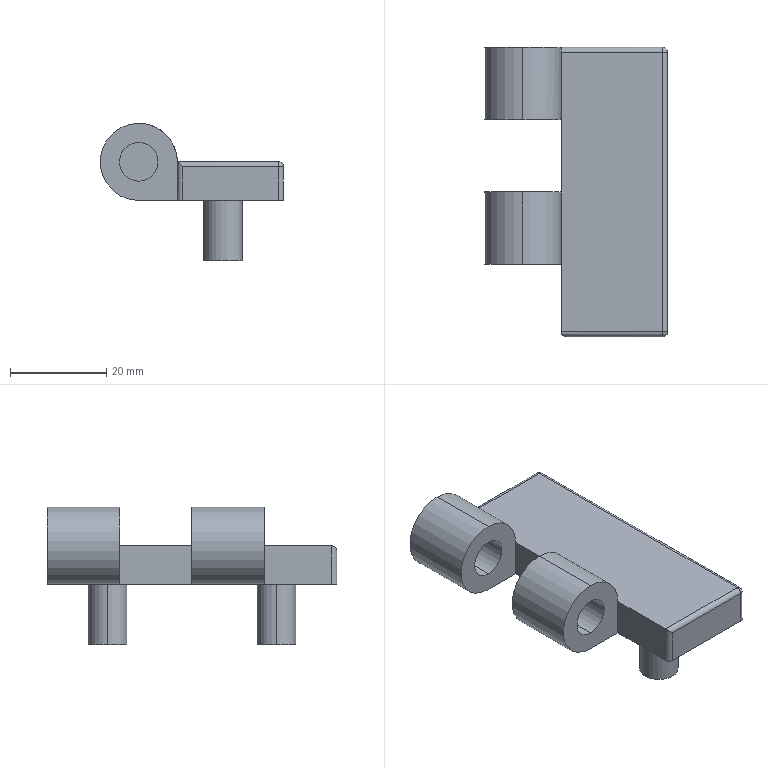Component | SolidWorks | DoorHinge1-1 | 1 solid | 33 faces | box 38 x 60 x 28.5 mm | volume 16826 mm3 | cylinder 18 | plane 13 | sphere 2 | commonest cylinder face diameters 8 x8 2 x6 16 x4
STEP:
#1=CARTESIAN_POINT('',(85.649,76.317,49.177));
#2=VERTEX_POINT('',#1);
#3=CARTESIAN_POINT('',(85.649,76.317,48.862));
#4=VERTEX_POINT('',#3);
#5=CARTESIAN_POINT('',(85.649,76.317,49.02));
#6=DIRECTION('',(-0.,-1.,0.));
#7=DIRECTION('',(0.,0.,-1.));
#8=AXIS2_PLACEMENT_3D('',#5,#6,#7);
#9=CIRCLE('',#8,0.1575);
#10=EDGE_CURVE('',#2,#4,#9,.T.);
#11=ORIENTED_EDGE('',*,*,#10,.F.);
#12=CARTESIAN_POINT('',(85.649,75.806,49.177));
#13=VERTEX_POINT('',#12);
#14=CARTESIAN_POINT('',(85.649,76.317,49.177));
#15=DIRECTION('',(-0.,-1.,0.));
#16=VECTOR('',#15,39.37);
#17=LINE('',#14,#16);
#18=EDGE_CURVE('',#2,#13,#17,.T.);
#19=ORIENTED_EDGE('',*,*,#18,.T.);
#20=CARTESIAN_POINT('',(85.649,75.806,48.862));
#21=VERTEX_POINT('',#20);
#22=CARTESIAN_POINT('',(85.649,75.806,49.02));
#23=DIRECTION('',(0.,1.,-0.));
#24=DIRECTION('',(-1.,0.,0.));
#25=AXIS2_PLACEMENT_3D('',#22,#23,#24);
#26=CIRCLE('',#25,0.1575);
#27=EDGE_CURVE('',#21,#13,#26,.T.);
#28=ORIENTED_EDGE('',*,*,#27,.F.);
#29=CARTESIAN_POINT('',(85.649,76.317,48.862));
#30=DIRECTION('',(-0.,-1.,0.));
#31=VECTOR('',#30,39.37);
#32=LINE('',#29,#31);
#33=EDGE_CURVE('',#4,#21,#32,.T.);
#34=ORIENTED_EDGE('',*,*,#33,.F.);
#35=EDGE_LOOP('',(#11,#19,#28,#34));
#36=FACE_OUTER_BOUND('',#35,.T.);
#37=CARTESIAN_POINT('',(85.649,76.317,49.02));
#38=DIRECTION('',(-0.,-1.,0.));
#39=DIRECTION('',(0.,0.,-1.));
#40=AXIS2_PLACEMENT_3D('',#37,#38,#39);
#41=CYLINDRICAL_SURFACE('',#40,0.1575);
#42=ADVANCED_FACE('',(#36),#41,.F.);
#43=CARTESIAN_POINT('',(86.495,75.904,48.213));
#44=VERTEX_POINT('',#43);
#45=CARTESIAN_POINT('',(86.18,75.904,48.213));
#46=VERTEX_POINT('',#45);
#47=CARTESIAN_POINT('',(86.338,75.904,48.213));
#48=DIRECTION('',(-0.,-0.,-1.));
#49=DIRECTION('',(1.,0.,0.));
#50=AXIS2_PLACEMENT_3D('',#47,#48,#49);
#51=CIRCLE('',#50,0.1575);
#52=EDGE_CURVE('',#44,#46,#51,.T.);
#53=ORIENTED_EDGE('',*,*,#52,.F.);
#54=CARTESIAN_POINT('',(86.495,75.904,48.705));
#55=VERTEX_POINT('',#54);
#56=CARTESIAN_POINT('',(86.495,75.904,48.213));
#57=DIRECTION('',(0.,0.,1.));
#58=VECTOR('',#57,39.37);
#59=LINE('',#56,#58);
#60=EDGE_CURVE('',#44,#55,#59,.T.);
#61=ORIENTED_EDGE('',*,*,#60,.T.);
#62=CARTESIAN_POINT('',(86.18,75.904,48.705));
#63=VERTEX_POINT('',#62);
#64=CARTESIAN_POINT('',(86.338,75.904,48.705));
#65=DIRECTION('',(-0.,-0.,-1.));
#66=DIRECTION('',(-1.,0.,0.));
#67=AXIS2_PLACEMENT_3D('',#64,#65,#66);
#68=CIRCLE('',#67,0.1575);
#69=EDGE_CURVE('',#55,#63,#68,.T.);
#70=ORIENTED_EDGE('',*,*,#69,.T.);
#71=CARTESIAN_POINT('',(86.18,75.904,48.213));
#72=DIRECTION('',(0.,0.,1.));
#73=VECTOR('',#72,39.37);
#74=LINE('',#71,#73);
#75=EDGE_CURVE('',#46,#63,#74,.T.);
#76=ORIENTED_EDGE('',*,*,#75,.F.);
#77=EDGE_LOOP('',(#53,#61,#70,#76));
#78=FACE_OUTER_BOUND('',#77,.T.);
#79=CARTESIAN_POINT('',(86.338,75.904,48.213));
#80=DIRECTION('',(0.,0.,1.));
#81=DIRECTION('',(-1.,0.,0.));
#82=AXIS2_PLACEMENT_3D('',#79,#80,#81);
#83=CYLINDRICAL_SURFACE('',#82,0.1575);
#84=ADVANCED_FACE('',(#78),#83,.T.);
#85=CARTESIAN_POINT('',(86.495,74.526,48.213));
#86=VERTEX_POINT('',#85);
#87=CARTESIAN_POINT('',(86.18,74.526,48.213));
#88=VERTEX_POINT('',#87);
#89=CARTESIAN_POINT('',(86.338,74.526,48.213));
#90=DIRECTION('',(-0.,-0.,-1.));
#91=DIRECTION('',(1.,0.,0.));
#92=AXIS2_PLACEMENT_3D('',#89,#90,#91);
#93=CIRCLE('',#92,0.1575);
#94=EDGE_CURVE('',#86,#88,#93,.T.);
#95=ORIENTED_EDGE('',*,*,#94,.F.);
#96=CARTESIAN_POINT('',(86.495,74.526,48.705));
#97=VERTEX_POINT('',#96);
#98=CARTESIAN_POINT('',(86.495,74.526,48.213));
#99=DIRECTION('',(0.,0.,1.));
#100=VECTOR('',#99,39.37);
#101=LINE('',#98,#100);
#102=EDGE_CURVE('',#86,#97,#101,.T.);
#103=ORIENTED_EDGE('',*,*,#102,.T.);
#104=CARTESIAN_POINT('',(86.18,74.526,48.705));
#105=VERTEX_POINT('',#104);
#106=CARTESIAN_POINT('',(86.338,74.526,48.705));
#107=DIRECTION('',(-0.,-0.,-1.));
#108=DIRECTION('',(-1.,0.,0.));
#109=AXIS2_PLACEMENT_3D('',#106,#107,#108);
#110=CIRCLE('',#109,0.1575);
#111=EDGE_CURVE('',#97,#105,#110,.T.);
#112=ORIENTED_EDGE('',*,*,#111,.T.);
#113=CARTESIAN_POINT('',(86.18,74.526,48.213));
#114=DIRECTION('',(0.,0.,1.));
#115=VECTOR('',#114,39.37);
#116=LINE('',#113,#115);
#117=EDGE_CURVE('',#88,#105,#116,.T.);
#118=ORIENTED_EDGE('',*,*,#117,.F.);
#119=EDGE_LOOP('',(#95,#103,#112,#118));
#120=FACE_OUTER_BOUND('',#119,.T.);
#121=CARTESIAN_POINT('',(86.338,74.526,48.213));
#122=DIRECTION('',(0.,0.,1.));
#123=DIRECTION('',(-1.,0.,0.));
#124=AXIS2_PLACEMENT_3D('',#121,#122,#123);
#125=CYLINDRICAL_SURFACE('',#124,0.1575);
#126=ADVANCED_FACE('',(#120),#125,.T.);
#127=CARTESIAN_POINT('',(85.649,75.215,49.177));
#128=VERTEX_POINT('',#127);
#129=CARTESIAN_POINT('',(85.649,75.215,48.862));
#130=VERTEX_POINT('',#129);
#131=CARTESIAN_POINT('',(85.649,75.215,49.02));
#132=DIRECTION('',(-0.,-1.,0.));
#133=DIRECTION('',(1.,0.,0.));
#134=AXIS2_PLACEMENT_3D('',#131,#132,#133);
#135=CIRCLE('',#134,0.1575);
#136=EDGE_CURVE('',#128,#130,#135,.T.);
#137=ORIENTED_EDGE('',*,*,#136,.F.);
#138=CARTESIAN_POINT('',(85.649,74.624,49.177));
#139=VERTEX_POINT('',#138);
#140=CARTESIAN_POINT('',(85.649,76.317,49.177));
#141=DIRECTION('',(-0.,-1.,0.));
#142=VECTOR('',#141,39.37);
#143=LINE('',#140,#142);
#144=EDGE_CURVE('',#128,#139,#143,.T.);
#145=ORIENTED_EDGE('',*,*,#144,.T.);
#146=CARTESIAN_POINT('',(85.649,74.624,48.862));
#147=VERTEX_POINT('',#146);
#148=CARTESIAN_POINT('',(85.649,74.624,49.02));
#149=DIRECTION('',(0.,1.,-0.));
#150=DIRECTION('',(0.,0.,-1.));
#151=AXIS2_PLACEMENT_3D('',#148,#149,#150);
#152=CIRCLE('',#151,0.1575);
#153=EDGE_CURVE('',#147,#139,#152,.T.);
#154=ORIENTED_EDGE('',*,*,#153,.F.);
#155=CARTESIAN_POINT('',(85.649,76.317,48.862));
#156=DIRECTION('',(-0.,-1.,0.));
#157=VECTOR('',#156,39.37);
#158=LINE('',#155,#157);
#159=EDGE_CURVE('',#130,#147,#158,.T.);
#160=ORIENTED_EDGE('',*,*,#159,.F.);
#161=EDGE_LOOP('',(#137,#145,#154,#160));
#162=FACE_OUTER_BOUND('',#161,.T.);
#163=CARTESIAN_POINT('',(85.649,76.317,49.02));
#164=DIRECTION('',(-0.,-1.,0.));
#165=DIRECTION('',(0.,0.,-1.));
#166=AXIS2_PLACEMENT_3D('',#163,#164,#165);
#167=CYLINDRICAL_SURFACE('',#166,0.1575);
#168=ADVANCED_FACE('',(#162),#167,.F.);
#169=CARTESIAN_POINT('',(85.649,75.806,49.335));
#170=VERTEX_POINT('',#169);
#171=CARTESIAN_POINT('',(85.649,75.806,48.705));
#172=VERTEX_POINT('',#171);
#173=CARTESIAN_POINT('',(85.649,75.806,49.02));
#174=DIRECTION('',(-0.,-1.,0.));
#175=DIRECTION('',(-1.,0.,0.));
#176=AXIS2_PLACEMENT_3D('',#173,#174,#175);
#177=CIRCLE('',#176,0.315);
#178=EDGE_CURVE('',#170,#172,#177,.T.);
#179=ORIENTED_EDGE('',*,*,#178,.F.);
#180=CARTESIAN_POINT('',(85.649,76.396,49.335));
#181=VERTEX_POINT('',#180);
#182=CARTESIAN_POINT('',(85.649,74.034,49.335));
#183=DIRECTION('',(0.,1.,-0.));
#184=VECTOR('',#183,39.37);
#185=LINE('',#182,#184);
#186=EDGE_CURVE('',#170,#181,#185,.T.);
#187=ORIENTED_EDGE('',*,*,#186,.T.);
#188=CARTESIAN_POINT('',(85.649,76.396,48.705));
#189=VERTEX_POINT('',#188);
#190=CARTESIAN_POINT('',(85.649,76.396,49.02));
#191=DIRECTION('',(-0.,-1.,0.));
#192=DIRECTION('',(0.,0.,-1.));
#193=AXIS2_PLACEMENT_3D('',#190,#191,#192);
#194=CIRCLE('',#193,0.315);
#195=EDGE_CURVE('',#181,#189,#194,.T.);
#196=ORIENTED_EDGE('',*,*,#195,.T.);
#197=CARTESIAN_POINT('',(85.649,74.034,48.705));
#198=DIRECTION('',(0.,1.,-0.));
#199=VECTOR('',#198,39.37);
#200=LINE('',#197,#199);
#201=EDGE_CURVE('',#172,#189,#200,.T.);
#202=ORIENTED_EDGE('',*,*,#201,.F.);
#203=EDGE_LOOP('',(#179,#187,#196,#202));
#204=FACE_OUTER_BOUND('',#203,.T.);
#205=CARTESIAN_POINT('',(85.649,74.034,49.02));
#206=DIRECTION('',(0.,1.,-0.));
#207=DIRECTION('',(0.,0.,1.));
#208=AXIS2_PLACEMENT_3D('',#205,#206,#207);
#209=CYLINDRICAL_SURFACE('',#208,0.315);
#210=ADVANCED_FACE('',(#204),#209,.T.);
#211=CARTESIAN_POINT('',(85.649,74.624,49.335));
#212=VERTEX_POINT('',#211);
#213=CARTESIAN_POINT('',(85.649,74.624,48.705));
#214=VERTEX_POINT('',#213);
#215=CARTESIAN_POINT('',(85.649,74.624,49.02));
#216=DIRECTION('',(-0.,-1.,0.));
#217=DIRECTION('',(0.,0.,-1.));
#218=AXIS2_PLACEMENT_3D('',#215,#216,#217);
#219=CIRCLE('',#218,0.315);
#220=EDGE_CURVE('',#212,#214,#219,.T.);
#221=ORIENTED_EDGE('',*,*,#220,.F.);
#222=CARTESIAN_POINT('',(85.649,75.215,49.335));
#223=VERTEX_POINT('',#222);
#224=CARTESIAN_POINT('',(85.649,74.034,49.335));
#225=DIRECTION('',(0.,1.,-0.));
#226=VECTOR('',#225,39.37);
#227=LINE('',#224,#226);
#228=EDGE_CURVE('',#212,#223,#227,.T.);
#229=ORIENTED_EDGE('',*,*,#228,.T.);
#230=CARTESIAN_POINT('',(85.649,75.215,48.705));
#231=VERTEX_POINT('',#230);
#232=CARTESIAN_POINT('',(85.649,75.215,49.02));
#233=DIRECTION('',(0.,1.,-0.));
#234=DIRECTION('',(1.,0.,0.));
#235=AXIS2_PLACEMENT_3D('',#232,#233,#234);
#236=CIRCLE('',#235,0.315);
#237=EDGE_CURVE('',#231,#223,#236,.T.);
#238=ORIENTED_EDGE('',*,*,#237,.F.);
#239=CARTESIAN_POINT('',(85.649,74.034,48.705));
#240=DIRECTION('',(0.,1.,-0.));
#241=VECTOR('',#240,39.37);
#242=LINE('',#239,#241);
#243=EDGE_CURVE('',#214,#231,#242,.T.);
#244=ORIENTED_EDGE('',*,*,#243,.F.);
#245=EDGE_LOOP('',(#221,#229,#238,#244));
#246=FACE_OUTER_BOUND('',#245,.T.);
#247=CARTESIAN_POINT('',(85.649,74.034,49.02));
#248=DIRECTION('',(0.,1.,-0.));
#249=DIRECTION('',(0.,0.,1.));
#250=AXIS2_PLACEMENT_3D('',#247,#248,#249);
#251=CYLINDRICAL_SURFACE('',#250,0.315);
#252=ADVANCED_FACE('',(#246),#251,.T.);
#253=CARTESIAN_POINT('',(86.338,74.526,48.705));
#254=DIRECTION('',(-0.,-0.,-1.));
#255=DIRECTION('',(-1.,0.,0.));
#256=AXIS2_PLACEMENT_3D('',#253,#254,#255);
#257=CIRCLE('',#256,0.1575);
#258=EDGE_CURVE('',#105,#97,#257,.T.);
#259=ORIENTED_EDGE('',*,*,#258,.F.);
#260=ORIENTED_EDGE('',*,*,#111,.F.);
#261=EDGE_LOOP('',(#259,#260));
#262=FACE_BOUND('',#261,.T.);
#263=CARTESIAN_POINT('',(86.338,75.904,48.705));
#264=DIRECTION('',(-0.,-0.,-1.));
#265=DIRECTION('',(-1.,0.,0.));
#266=AXIS2_PLACEMENT_3D('',#263,#264,#265);
#267=CIRCLE('',#266,0.1575);
#268=EDGE_CURVE('',#63,#55,#267,.T.);
#269=ORIENTED_EDGE('',*,*,#268,.F.);
#270=ORIENTED_EDGE('',*,*,#69,.F.);
#271=EDGE_LOOP('',(#269,#270));
#272=FACE_BOUND('',#271,.T.);
#273=CARTESIAN_POINT('',(86.79,76.396,48.705));
#274=VERTEX_POINT('',#273);
#275=CARTESIAN_POINT('',(84.813,76.396,48.705));
#276=DIRECTION('',(1.,-0.,-0.));
#277=VECTOR('',#276,39.37);
#278=LINE('',#275,#277);
#279=EDGE_CURVE('',#189,#274,#278,.T.);
#280=ORIENTED_EDGE('',*,*,#279,.T.);
#281=CARTESIAN_POINT('',(86.83,76.357,48.705));
#282=VERTEX_POINT('',#281);
#283=CARTESIAN_POINT('',(86.79,76.357,48.705));
#284=DIRECTION('',(-0.,-0.,-1.));
#285=DIRECTION('',(-1.,0.,0.));
#286=AXIS2_PLACEMENT_3D('',#283,#284,#285);
#287=CIRCLE('',#286,0.03937);
#288=EDGE_CURVE('',#274,#282,#287,.T.);
#289=ORIENTED_EDGE('',*,*,#288,.T.);
#290=CARTESIAN_POINT('',(86.83,74.073,48.705));
#291=VERTEX_POINT('',#290);
#292=CARTESIAN_POINT('',(86.83,74.034,48.705));
#293=DIRECTION('',(0.,1.,-0.));
#294=VECTOR('',#293,39.37);
#295=LINE('',#292,#294);
#296=EDGE_CURVE('',#291,#282,#295,.T.);
#297=ORIENTED_EDGE('',*,*,#296,.F.);
#298=CARTESIAN_POINT('',(86.79,74.034,48.705));
#299=VERTEX_POINT('',#298);
#300=CARTESIAN_POINT('',(86.79,74.073,48.705));
#301=DIRECTION('',(-0.,-0.,-1.));
#302=DIRECTION('',(-1.,0.,0.));
#303=AXIS2_PLACEMENT_3D('',#300,#301,#302);
#304=CIRCLE('',#303,0.03937);
#305=EDGE_CURVE('',#291,#299,#304,.T.);
#306=ORIENTED_EDGE('',*,*,#305,.T.);
#307=CARTESIAN_POINT('',(86.003,74.034,48.705));
#308=VERTEX_POINT('',#307);
#309=CARTESIAN_POINT('',(84.813,74.034,48.705));
#310=DIRECTION('',(1.,-0.,-0.));
#311=VECTOR('',#310,39.37);
#312=LINE('',#309,#311);
#313=EDGE_CURVE('',#308,#299,#312,.T.);
#314=ORIENTED_EDGE('',*,*,#313,.F.);
#315=CARTESIAN_POINT('',(85.963,74.073,48.705));
#316=VERTEX_POINT('',#315);
#317=CARTESIAN_POINT('',(86.003,74.073,48.705));
#318=DIRECTION('',(-0.,-0.,-1.));
#319=DIRECTION('',(-1.,0.,0.));
#320=AXIS2_PLACEMENT_3D('',#317,#318,#319);
#321=CIRCLE('',#320,0.03937);
#322=EDGE_CURVE('',#308,#316,#321,.T.);
#323=ORIENTED_EDGE('',*,*,#322,.T.);
#324=CARTESIAN_POINT('',(85.963,74.624,48.705));
#325=VERTEX_POINT('',#324);
#326=CARTESIAN_POINT('',(85.963,77.404,48.705));
#327=DIRECTION('',(0.,1.,-0.));
#328=VECTOR('',#327,39.37);
#329=LINE('',#326,#328);
#330=EDGE_CURVE('',#316,#325,#329,.T.);
#331=ORIENTED_EDGE('',*,*,#330,.T.);
#332=CARTESIAN_POINT('',(86.136,74.624,48.705));
#333=DIRECTION('',(-1.,0.,0.));
#334=VECTOR('',#333,39.37);
#335=LINE('',#332,#334);
#336=EDGE_CURVE('',#325,#214,#335,.T.);
#337=ORIENTED_EDGE('',*,*,#336,.T.);
#338=ORIENTED_EDGE('',*,*,#243,.T.);
#339=CARTESIAN_POINT('',(85.963,75.215,48.705));
#340=VERTEX_POINT('',#339);
#341=CARTESIAN_POINT('',(85.334,75.215,48.705));
#342=DIRECTION('',(1.,-0.,-0.));
#343=VECTOR('',#342,39.37);
#344=LINE('',#341,#343);
#345=EDGE_CURVE('',#231,#340,#344,.T.);
#346=ORIENTED_EDGE('',*,*,#345,.T.);
#347=CARTESIAN_POINT('',(85.963,75.806,48.705));
#348=VERTEX_POINT('',#347);
#349=CARTESIAN_POINT('',(85.963,75.215,48.705));
#350=DIRECTION('',(0.,1.,-0.));
#351=VECTOR('',#350,39.37);
#352=LINE('',#349,#351);
#353=EDGE_CURVE('',#340,#348,#352,.T.);
#354=ORIENTED_EDGE('',*,*,#353,.T.);
#355=CARTESIAN_POINT('',(85.963,75.806,48.705));
#356=DIRECTION('',(-1.,0.,0.));
#357=VECTOR('',#356,39.37);
#358=LINE('',#355,#357);
#359=EDGE_CURVE('',#348,#172,#358,.T.);
#360=ORIENTED_EDGE('',*,*,#359,.T.);
#361=ORIENTED_EDGE('',*,*,#201,.T.);
#362=EDGE_LOOP('',(#280,#289,#297,#306,#314,#323,#331,#337,#338,#346,#354,#360,#361));
#363=FACE_OUTER_BOUND('',#362,.T.);
#364=CARTESIAN_POINT('',(84.813,74.034,48.705));
#365=DIRECTION('',(0.,0.,1.));
#366=DIRECTION('',(-1.,0.,0.));
#367=AXIS2_PLACEMENT_3D('',#364,#365,#366);
#368=PLANE('',#367);
#369=ADVANCED_FACE('',(#262,#272,#363),#368,.F.);
#370=ORIENTED_EDGE('',*,*,#228,.F.);
#371=CARTESIAN_POINT('',(85.963,74.624,49.02));
#372=VERTEX_POINT('',#371);
#373=CARTESIAN_POINT('',(85.649,74.624,49.02));
#374=DIRECTION('',(-0.,-1.,0.));
#375=DIRECTION('',(0.,0.,-1.));
#376=AXIS2_PLACEMENT_3D('',#373,#374,#375);
#377=CIRCLE('',#376,0.315);
#378=EDGE_CURVE('',#372,#212,#377,.T.);
#379=ORIENTED_EDGE('',*,*,#378,.F.);
#380=CARTESIAN_POINT('',(85.963,75.215,49.02));
#381=VERTEX_POINT('',#380);
#382=CARTESIAN_POINT('',(85.963,74.034,49.02));
#383=DIRECTION('',(0.,1.,-0.));
#384=VECTOR('',#383,39.37);
#385=LINE('',#382,#384);
#386=EDGE_CURVE('',#372,#381,#385,.T.);
#387=ORIENTED_EDGE('',*,*,#386,.T.);
#388=CARTESIAN_POINT('',(85.649,75.215,49.02));
#389=DIRECTION('',(0.,1.,-0.));
#390=DIRECTION('',(1.,0.,0.));
#391=AXIS2_PLACEMENT_3D('',#388,#389,#390);
#392=CIRCLE('',#391,0.315);
#393=EDGE_CURVE('',#223,#381,#392,.T.);
#394=ORIENTED_EDGE('',*,*,#393,.F.);
#395=EDGE_LOOP('',(#370,#379,#387,#394));
#396=FACE_OUTER_BOUND('',#395,.T.);
#397=CARTESIAN_POINT('',(85.649,74.034,49.02));
#398=DIRECTION('',(0.,1.,-0.));
#399=DIRECTION('',(0.,0.,1.));
#400=AXIS2_PLACEMENT_3D('',#397,#398,#399);
#401=CYLINDRICAL_SURFACE('',#400,0.315);
#402=ADVANCED_FACE('',(#396),#401,.T.);
#403=ORIENTED_EDGE('',*,*,#186,.F.);
#404=CARTESIAN_POINT('',(85.963,75.806,49.02));
#405=VERTEX_POINT('',#404);
#406=CARTESIAN_POINT('',(85.649,75.806,49.02));
#407=DIRECTION('',(-0.,-1.,0.));
#408=DIRECTION('',(-1.,0.,0.));
#409=AXIS2_PLACEMENT_3D('',#406,#407,#408);
#410=CIRCLE('',#409,0.315);
#411=EDGE_CURVE('',#405,#170,#410,.T.);
#412=ORIENTED_EDGE('',*,*,#411,.F.);
#413=CARTESIAN_POINT('',(85.963,76.357,49.02));
#414=VERTEX_POINT('',#413);
#415=CARTESIAN_POINT('',(85.963,74.034,49.02));
#416=DIRECTION('',(0.,1.,-0.));
#417=VECTOR('',#416,39.37);
#418=LINE('',#415,#417);
#419=EDGE_CURVE('',#405,#414,#418,.T.);
#420=ORIENTED_EDGE('',*,*,#419,.T.);
#421=CARTESIAN_POINT('',(85.961,76.396,48.981));
#422=VERTEX_POINT('',#421);
#423=CARTESIAN_POINT('',(85.963,76.357,49.02));
#424=CARTESIAN_POINT('',(85.963,76.362,49.02));
#425=CARTESIAN_POINT('',(85.963,76.367,49.019));
#426=CARTESIAN_POINT('',(85.963,76.377,49.015));
#427=CARTESIAN_POINT('',(85.963,76.381,49.012));
#428=CARTESIAN_POINT('',(85.963,76.388,49.005));
#429=CARTESIAN_POINT('',(85.963,76.391,49.));
#430=CARTESIAN_POINT('',(85.962,76.395,48.991));
#431=CARTESIAN_POINT('',(85.962,76.396,48.986));
#432=CARTESIAN_POINT('',(85.961,76.396,48.981));
#433=B_SPLINE_CURVE_WITH_KNOTS('',3,(#423,#424,#425,#426,#427,#428,#429,#430,#431,#432),.UNSPECIFIED.,.F.,.F.,(4,2,2,2,4),(0.,0.0003912,0.0007823,0.001173,0.001565),.UNSPECIFIED.);
#434=EDGE_CURVE('',#414,#422,#433,.T.);
#435=ORIENTED_EDGE('',*,*,#434,.T.);
#436=CARTESIAN_POINT('',(85.649,76.396,49.02));
#437=DIRECTION('',(-0.,-1.,0.));
#438=DIRECTION('',(0.,0.,-1.));
#439=AXIS2_PLACEMENT_3D('',#436,#437,#438);
#440=CIRCLE('',#439,0.315);
#441=EDGE_CURVE('',#422,#181,#440,.T.);
#442=ORIENTED_EDGE('',*,*,#441,.T.);
#443=EDGE_LOOP('',(#403,#412,#420,#435,#442));
#444=FACE_OUTER_BOUND('',#443,.T.);
#445=CARTESIAN_POINT('',(85.649,74.034,49.02));
#446=DIRECTION('',(0.,1.,-0.));
#447=DIRECTION('',(0.,0.,1.));
#448=AXIS2_PLACEMENT_3D('',#445,#446,#447);
#449=CYLINDRICAL_SURFACE('',#448,0.315);
#450=ADVANCED_FACE('',(#444),#449,.T.);
#451=ORIENTED_EDGE('',*,*,#144,.F.);
#452=CARTESIAN_POINT('',(85.649,75.215,49.02));
#453=DIRECTION('',(-0.,-1.,0.));
#454=DIRECTION('',(1.,0.,0.));
#455=AXIS2_PLACEMENT_3D('',#452,#453,#454);
#456=CIRCLE('',#455,0.1575);
#457=EDGE_CURVE('',#130,#128,#456,.T.);
#458=ORIENTED_EDGE('',*,*,#457,.F.);
#459=ORIENTED_EDGE('',*,*,#159,.T.);
#460=CARTESIAN_POINT('',(85.649,74.624,49.02));
#461=DIRECTION('',(0.,1.,-0.));
#462=DIRECTION('',(0.,0.,-1.));
#463=AXIS2_PLACEMENT_3D('',#460,#461,#462);
#464=CIRCLE('',#463,0.1575);
#465=EDGE_CURVE('',#139,#147,#464,.T.);
#466=ORIENTED_EDGE('',*,*,#465,.F.);
#467=EDGE_LOOP('',(#451,#458,#459,#466));
#468=FACE_OUTER_BOUND('',#467,.T.);
#469=CARTESIAN_POINT('',(85.649,76.317,49.02));
#470=DIRECTION('',(-0.,-1.,0.));
#471=DIRECTION('',(0.,0.,-1.));
#472=AXIS2_PLACEMENT_3D('',#469,#470,#471);
#473=CYLINDRICAL_SURFACE('',#472,0.1575);
#474=ADVANCED_FACE('',(#468),#473,.F.);
#475=CARTESIAN_POINT('',(86.79,74.034,48.981));
#476=VERTEX_POINT('',#475);
#477=CARTESIAN_POINT('',(86.003,74.034,48.981));
#478=VERTEX_POINT('',#477);
#479=CARTESIAN_POINT('',(85.963,74.034,48.981));
#480=DIRECTION('',(-1.,0.,0.));
#481=VECTOR('',#480,39.37);
#482=LINE('',#479,#481);
#483=EDGE_CURVE('',#476,#478,#482,.T.);
#484=ORIENTED_EDGE('',*,*,#483,.T.);
#485=CARTESIAN_POINT('',(86.003,74.034,49.02));
#486=DIRECTION('',(-0.,-0.,-1.));
#487=VECTOR('',#486,39.37);
#488=LINE('',#485,#487);
#489=EDGE_CURVE('',#478,#308,#488,.T.);
#490=ORIENTED_EDGE('',*,*,#489,.T.);
#491=ORIENTED_EDGE('',*,*,#313,.T.);
#492=CARTESIAN_POINT('',(86.79,74.034,49.02));
#493=DIRECTION('',(0.,0.,1.));
#494=VECTOR('',#493,39.37);
#495=LINE('',#492,#494);
#496=EDGE_CURVE('',#299,#476,#495,.T.);
#497=ORIENTED_EDGE('',*,*,#496,.T.);
#498=EDGE_LOOP('',(#484,#490,#491,#497));
#499=FACE_OUTER_BOUND('',#498,.T.);
#500=CARTESIAN_POINT('',(84.813,74.034,49.02));
#501=DIRECTION('',(-0.,-1.,0.));
#502=DIRECTION('',(-0.,-0.,-1.));
#503=AXIS2_PLACEMENT_3D('',#500,#501,#502);
#504=PLANE('',#503);
#505=ADVANCED_FACE('',(#499),#504,.T.);
#506=ORIENTED_EDGE('',*,*,#296,.T.);
#507=CARTESIAN_POINT('',(86.83,76.357,48.981));
#508=VERTEX_POINT('',#507);
#509=CARTESIAN_POINT('',(86.83,76.357,49.02));
#510=DIRECTION('',(0.,0.,1.));
#511=VECTOR('',#510,39.37);
#512=LINE('',#509,#511);
#513=EDGE_CURVE('',#282,#508,#512,.T.);
#514=ORIENTED_EDGE('',*,*,#513,.T.);
#515=CARTESIAN_POINT('',(86.83,74.073,48.981));
#516=VERTEX_POINT('',#515);
#517=CARTESIAN_POINT('',(86.83,74.034,48.981));
#518=DIRECTION('',(-0.,-1.,0.));
#519=VECTOR('',#518,39.37);
#520=LINE('',#517,#519);
#521=EDGE_CURVE('',#508,#516,#520,.T.);
#522=ORIENTED_EDGE('',*,*,#521,.T.);
#523=CARTESIAN_POINT('',(86.83,74.073,48.705));
#524=DIRECTION('',(-0.,-0.,-1.));
#525=VECTOR('',#524,39.37);
#526=LINE('',#523,#525);
#527=EDGE_CURVE('',#516,#291,#526,.T.);
#528=ORIENTED_EDGE('',*,*,#527,.T.);
#529=EDGE_LOOP('',(#506,#514,#522,#528));
#530=FACE_OUTER_BOUND('',#529,.T.);
#531=CARTESIAN_POINT('',(86.83,74.034,49.02));
#532=DIRECTION('',(-1.,0.,0.));
#533=DIRECTION('',(-0.,-0.,-1.));
#534=AXIS2_PLACEMENT_3D('',#531,#532,#533);
#535=PLANE('',#534);
#536=ADVANCED_FACE('',(#530),#535,.F.);
#537=CARTESIAN_POINT('',(85.963,74.073,49.02));
#538=VERTEX_POINT('',#537);
#539=CARTESIAN_POINT('',(85.963,74.034,49.02));
#540=DIRECTION('',(0.,1.,-0.));
#541=VECTOR('',#540,39.37);
#542=LINE('',#539,#541);
#543=EDGE_CURVE('',#538,#372,#542,.T.);
#544=ORIENTED_EDGE('',*,*,#543,.F.);
#545=CARTESIAN_POINT('',(86.79,74.073,49.02));
#546=VERTEX_POINT('',#545);
#547=CARTESIAN_POINT('',(86.83,74.073,49.02));
#548=DIRECTION('',(1.,-0.,-0.));
#549=VECTOR('',#548,39.37);
#550=LINE('',#547,#549);
#551=EDGE_CURVE('',#538,#546,#550,.T.);
#552=ORIENTED_EDGE('',*,*,#551,.T.);
#553=CARTESIAN_POINT('',(86.79,76.357,49.02));
#554=VERTEX_POINT('',#553);
#555=CARTESIAN_POINT('',(86.79,74.034,49.02));
#556=DIRECTION('',(0.,1.,-0.));
#557=VECTOR('',#556,39.37);
#558=LINE('',#555,#557);
#559=EDGE_CURVE('',#546,#554,#558,.T.);
#560=ORIENTED_EDGE('',*,*,#559,.T.);
#561=CARTESIAN_POINT('',(84.813,76.357,49.02));
#562=DIRECTION('',(-1.,0.,0.));
#563=VECTOR('',#562,39.37);
#564=LINE('',#561,#563);
#565=EDGE_CURVE('',#554,#414,#564,.T.);
#566=ORIENTED_EDGE('',*,*,#565,.T.);
#567=ORIENTED_EDGE('',*,*,#419,.F.);
#568=CARTESIAN_POINT('',(85.963,74.034,49.02));
#569=DIRECTION('',(0.,1.,-0.));
#570=VECTOR('',#569,39.37);
#571=LINE('',#568,#570);
#572=EDGE_CURVE('',#381,#405,#571,.T.);
#573=ORIENTED_EDGE('',*,*,#572,.F.);
#574=ORIENTED_EDGE('',*,*,#386,.F.);
#575=EDGE_LOOP('',(#544,#552,#560,#566,#567,#573,#574));
#576=FACE_OUTER_BOUND('',#575,.T.);
#577=CARTESIAN_POINT('',(84.813,74.034,49.02));
#578=DIRECTION('',(-0.,0.,-1.));
#579=DIRECTION('',(1.,-0.,-0.));
#580=AXIS2_PLACEMENT_3D('',#577,#578,#579);
#581=PLANE('',#580);
#582=ADVANCED_FACE('',(#576),#581,.F.);
#583=CARTESIAN_POINT('',(86.79,76.396,48.981));
#584=VERTEX_POINT('',#583);
#585=CARTESIAN_POINT('',(84.813,76.396,48.981));
#586=DIRECTION('',(1.,-0.,-0.));
#587=VECTOR('',#586,39.37);
#588=LINE('',#585,#587);
#589=EDGE_CURVE('',#422,#584,#588,.T.);
#590=ORIENTED_EDGE('',*,*,#589,.T.);
#591=CARTESIAN_POINT('',(86.79,76.396,49.02));
#592=DIRECTION('',(-0.,-0.,-1.));
#593=VECTOR('',#592,39.37);
#594=LINE('',#591,#593);
#595=EDGE_CURVE('',#584,#274,#594,.T.);
#596=ORIENTED_EDGE('',*,*,#595,.T.);
#597=ORIENTED_EDGE('',*,*,#279,.F.);
#598=ORIENTED_EDGE('',*,*,#195,.F.);
#599=ORIENTED_EDGE('',*,*,#441,.F.);
#600=EDGE_LOOP('',(#590,#596,#597,#598,#599));
#601=FACE_OUTER_BOUND('',#600,.T.);
#602=CARTESIAN_POINT('',(84.813,76.396,49.02));
#603=DIRECTION('',(-0.,-1.,0.));
#604=DIRECTION('',(-0.,-0.,-1.));
#605=AXIS2_PLACEMENT_3D('',#602,#603,#604);
#606=PLANE('',#605);
#607=ADVANCED_FACE('',(#601),#606,.F.);
#608=ORIENTED_EDGE('',*,*,#102,.F.);
#609=CARTESIAN_POINT('',(86.338,74.526,48.213));
#610=DIRECTION('',(-0.,-0.,-1.));
#611=DIRECTION('',(1.,0.,0.));
#612=AXIS2_PLACEMENT_3D('',#609,#610,#611);
#613=CIRCLE('',#612,0.1575);
#614=EDGE_CURVE('',#88,#86,#613,.T.);
#615=ORIENTED_EDGE('',*,*,#614,.F.);
#616=ORIENTED_EDGE('',*,*,#117,.T.);
#617=ORIENTED_EDGE('',*,*,#258,.T.);
#618=EDGE_LOOP('',(#608,#615,#616,#617));
#619=FACE_OUTER_BOUND('',#618,.T.);
#620=CARTESIAN_POINT('',(86.338,74.526,48.213));
#621=DIRECTION('',(0.,0.,1.));
#622=DIRECTION('',(-1.,0.,0.));
#623=AXIS2_PLACEMENT_3D('',#620,#621,#622);
#624=CYLINDRICAL_SURFACE('',#623,0.1575);
#625=ADVANCED_FACE('',(#619),#624,.T.);
#626=ORIENTED_EDGE('',*,*,#614,.T.);
#627=ORIENTED_EDGE('',*,*,#94,.T.);
#628=EDGE_LOOP('',(#626,#627));
#629=FACE_OUTER_BOUND('',#628,.T.);
#630=CARTESIAN_POINT('',(86.338,74.526,48.213));
#631=DIRECTION('',(-0.,-0.,-1.));
#632=DIRECTION('',(1.,-0.,-0.));
#633=AXIS2_PLACEMENT_3D('',#630,#631,#632);
#634=PLANE('',#633);
#635=ADVANCED_FACE('',(#629),#634,.T.);
#636=ORIENTED_EDGE('',*,*,#60,.F.);
#637=CARTESIAN_POINT('',(86.338,75.904,48.213));
#638=DIRECTION('',(-0.,-0.,-1.));
#639=DIRECTION('',(1.,0.,0.));
#640=AXIS2_PLACEMENT_3D('',#637,#638,#639);
#641=CIRCLE('',#640,0.1575);
#642=EDGE_CURVE('',#46,#44,#641,.T.);
#643=ORIENTED_EDGE('',*,*,#642,.F.);
#644=ORIENTED_EDGE('',*,*,#75,.T.);
#645=ORIENTED_EDGE('',*,*,#268,.T.);
#646=EDGE_LOOP('',(#636,#643,#644,#645));
#647=FACE_OUTER_BOUND('',#646,.T.);
#648=CARTESIAN_POINT('',(86.338,75.904,48.213));
#649=DIRECTION('',(0.,0.,1.));
#650=DIRECTION('',(-1.,0.,0.));
#651=AXIS2_PLACEMENT_3D('',#648,#649,#650);
#652=CYLINDRICAL_SURFACE('',#651,0.1575);
#653=ADVANCED_FACE('',(#647),#652,.T.);
#654=ORIENTED_EDGE('',*,*,#642,.T.);
#655=ORIENTED_EDGE('',*,*,#52,.T.);
#656=EDGE_LOOP('',(#654,#655));
#657=FACE_OUTER_BOUND('',#656,.T.);
#658=CARTESIAN_POINT('',(86.338,75.904,48.213));
#659=DIRECTION('',(-0.,-0.,-1.));
#660=DIRECTION('',(1.,-0.,-0.));
#661=AXIS2_PLACEMENT_3D('',#658,#659,#660);
#662=PLANE('',#661);
#663=ADVANCED_FACE('',(#657),#662,.T.);
#664=ORIENTED_EDGE('',*,*,#330,.F.);
#665=CARTESIAN_POINT('',(85.963,74.073,50.988));
#666=DIRECTION('',(0.,0.,1.));
#667=VECTOR('',#666,39.37);
#668=LINE('',#665,#667);
#669=EDGE_CURVE('',#316,#538,#668,.T.);
#670=ORIENTED_EDGE('',*,*,#669,.T.);
#671=ORIENTED_EDGE('',*,*,#543,.T.);
#672=CARTESIAN_POINT('',(85.963,74.624,50.988));
#673=DIRECTION('',(-0.,-0.,-1.));
#674=VECTOR('',#673,39.37);
#675=LINE('',#672,#674);
#676=EDGE_CURVE('',#372,#325,#675,.T.);
#677=ORIENTED_EDGE('',*,*,#676,.T.);
#678=EDGE_LOOP('',(#664,#670,#671,#677));
#679=FACE_OUTER_BOUND('',#678,.T.);
#680=CARTESIAN_POINT('',(85.963,77.404,50.988));
#681=DIRECTION('',(-1.,0.,0.));
#682=DIRECTION('',(-0.,-0.,-1.));
#683=AXIS2_PLACEMENT_3D('',#680,#681,#682);
#684=PLANE('',#683);
#685=ADVANCED_FACE('',(#679),#684,.T.);
#686=ORIENTED_EDGE('',*,*,#153,.T.);
#687=ORIENTED_EDGE('',*,*,#465,.T.);
#688=EDGE_LOOP('',(#686,#687));
#689=FACE_BOUND('',#688,.T.);
#690=ORIENTED_EDGE('',*,*,#378,.T.);
#691=ORIENTED_EDGE('',*,*,#220,.T.);
#692=ORIENTED_EDGE('',*,*,#336,.F.);
#693=ORIENTED_EDGE('',*,*,#676,.F.);
#694=EDGE_LOOP('',(#690,#691,#692,#693));
#695=FACE_OUTER_BOUND('',#694,.T.);
#696=CARTESIAN_POINT('',(86.136,74.624,50.988));
#697=DIRECTION('',(-0.,-1.,0.));
#698=DIRECTION('',(-0.,-0.,-1.));
#699=AXIS2_PLACEMENT_3D('',#696,#697,#698);
#700=PLANE('',#699);
#701=ADVANCED_FACE('',(#689,#695),#700,.T.);
#702=ORIENTED_EDGE('',*,*,#572,.T.);
#703=CARTESIAN_POINT('',(85.963,75.806,50.988));
#704=DIRECTION('',(-0.,-0.,-1.));
#705=VECTOR('',#704,39.37);
#706=LINE('',#703,#705);
#707=EDGE_CURVE('',#405,#348,#706,.T.);
#708=ORIENTED_EDGE('',*,*,#707,.T.);
#709=ORIENTED_EDGE('',*,*,#353,.F.);
#710=CARTESIAN_POINT('',(85.963,75.215,50.988));
#711=DIRECTION('',(-0.,-0.,-1.));
#712=VECTOR('',#711,39.37);
#713=LINE('',#710,#712);
#714=EDGE_CURVE('',#381,#340,#713,.T.);
#715=ORIENTED_EDGE('',*,*,#714,.F.);
#716=EDGE_LOOP('',(#702,#708,#709,#715));
#717=FACE_OUTER_BOUND('',#716,.T.);
#718=CARTESIAN_POINT('',(85.963,75.215,50.988));
#719=DIRECTION('',(-1.,0.,0.));
#720=DIRECTION('',(0.,1.,-0.));
#721=AXIS2_PLACEMENT_3D('',#718,#719,#720);
#722=PLANE('',#721);
#723=ADVANCED_FACE('',(#717),#722,.T.);
#724=ORIENTED_EDGE('',*,*,#457,.T.);
#725=ORIENTED_EDGE('',*,*,#136,.T.);
#726=EDGE_LOOP('',(#724,#725));
#727=FACE_BOUND('',#726,.T.);
#728=ORIENTED_EDGE('',*,*,#237,.T.);
#729=ORIENTED_EDGE('',*,*,#393,.T.);
#730=ORIENTED_EDGE('',*,*,#714,.T.);
#731=ORIENTED_EDGE('',*,*,#345,.F.);
#732=EDGE_LOOP('',(#728,#729,#730,#731));
#733=FACE_OUTER_BOUND('',#732,.T.);
#734=CARTESIAN_POINT('',(85.334,75.215,50.988));
#735=DIRECTION('',(0.,1.,-0.));
#736=DIRECTION('',(1.,-0.,-0.));
#737=AXIS2_PLACEMENT_3D('',#734,#735,#736);
#738=PLANE('',#737);
#739=ADVANCED_FACE('',(#727,#733),#738,.T.);
#740=ORIENTED_EDGE('',*,*,#27,.T.);
#741=CARTESIAN_POINT('',(85.649,75.806,49.02));
#742=DIRECTION('',(0.,1.,-0.));
#743=DIRECTION('',(-1.,0.,0.));
#744=AXIS2_PLACEMENT_3D('',#741,#742,#743);
#745=CIRCLE('',#744,0.1575);
#746=EDGE_CURVE('',#13,#21,#745,.T.);
#747=ORIENTED_EDGE('',*,*,#746,.T.);
#748=EDGE_LOOP('',(#740,#747));
#749=FACE_BOUND('',#748,.T.);
#750=ORIENTED_EDGE('',*,*,#411,.T.);
#751=ORIENTED_EDGE('',*,*,#178,.T.);
#752=ORIENTED_EDGE('',*,*,#359,.F.);
#753=ORIENTED_EDGE('',*,*,#707,.F.);
#754=EDGE_LOOP('',(#750,#751,#752,#753));
#755=FACE_OUTER_BOUND('',#754,.T.);
#756=CARTESIAN_POINT('',(85.963,75.806,50.988));
#757=DIRECTION('',(-0.,-1.,0.));
#758=DIRECTION('',(-1.,0.,0.));
#759=AXIS2_PLACEMENT_3D('',#756,#757,#758);
#760=PLANE('',#759);
#761=ADVANCED_FACE('',(#749,#755),#760,.T.);
#762=CARTESIAN_POINT('',(85.649,76.317,49.02));
#763=DIRECTION('',(-0.,-1.,0.));
#764=DIRECTION('',(0.,0.,-1.));
#765=AXIS2_PLACEMENT_3D('',#762,#763,#764);
#766=CIRCLE('',#765,0.1575);
#767=EDGE_CURVE('',#4,#2,#766,.T.);
#768=ORIENTED_EDGE('',*,*,#767,.T.);
#769=ORIENTED_EDGE('',*,*,#10,.T.);
#770=EDGE_LOOP('',(#768,#769));
#771=FACE_OUTER_BOUND('',#770,.T.);
#772=CARTESIAN_POINT('',(85.649,76.317,49.02));
#773=DIRECTION('',(-0.,-1.,0.));
#774=DIRECTION('',(-0.,-0.,-1.));
#775=AXIS2_PLACEMENT_3D('',#772,#773,#774);
#776=PLANE('',#775);
#777=ADVANCED_FACE('',(#771),#776,.T.);
#778=ORIENTED_EDGE('',*,*,#18,.F.);
#779=ORIENTED_EDGE('',*,*,#767,.F.);
#780=ORIENTED_EDGE('',*,*,#33,.T.);
#781=ORIENTED_EDGE('',*,*,#746,.F.);
#782=EDGE_LOOP('',(#778,#779,#780,#781));
#783=FACE_OUTER_BOUND('',#782,.T.);
#784=CARTESIAN_POINT('',(85.649,76.317,49.02));
#785=DIRECTION('',(-0.,-1.,0.));
#786=DIRECTION('',(0.,0.,-1.));
#787=AXIS2_PLACEMENT_3D('',#784,#785,#786);
#788=CYLINDRICAL_SURFACE('',#787,0.1575);
#789=ADVANCED_FACE('',(#783),#788,.F.);
#790=ORIENTED_EDGE('',*,*,#322,.F.);
#791=ORIENTED_EDGE('',*,*,#489,.F.);
#792=CARTESIAN_POINT('',(85.963,74.073,49.02));
#793=CARTESIAN_POINT('',(85.963,74.05,49.02));
#794=CARTESIAN_POINT('',(85.98,74.034,49.004));
#795=CARTESIAN_POINT('',(86.003,74.034,48.981));
#796=(BOUNDED_CURVE()B_SPLINE_CURVE(3,(#792,#793,#794,#795),.UNSPECIFIED.,.F.,.F.)B_SPLINE_CURVE_WITH_KNOTS((4,4),(3.142,4.712),.UNSPECIFIED.)CURVE()GEOMETRIC_REPRESENTATION_ITEM()RATIONAL_B_SPLINE_CURVE((1.,0.8047,0.8047,1.))REPRESENTATION_ITEM(''));
#797=EDGE_CURVE('',#538,#478,#796,.T.);
#798=ORIENTED_EDGE('',*,*,#797,.F.);
#799=ORIENTED_EDGE('',*,*,#669,.F.);
#800=EDGE_LOOP('',(#790,#791,#798,#799));
#801=FACE_OUTER_BOUND('',#800,.T.);
#802=CARTESIAN_POINT('',(86.003,74.073,49.02));
#803=DIRECTION('',(-0.,-0.,-1.));
#804=DIRECTION('',(1.,0.,0.));
#805=AXIS2_PLACEMENT_3D('',#802,#803,#804);
#806=CYLINDRICAL_SURFACE('',#805,0.03937);
#807=ADVANCED_FACE('',(#801),#806,.T.);
#808=ORIENTED_EDGE('',*,*,#305,.F.);
#809=ORIENTED_EDGE('',*,*,#527,.F.);
#810=CARTESIAN_POINT('',(86.79,74.073,48.981));
#811=DIRECTION('',(0.,0.,1.));
#812=DIRECTION('',(-1.,0.,0.));
#813=AXIS2_PLACEMENT_3D('',#810,#811,#812);
#814=CIRCLE('',#813,0.03937);
#815=EDGE_CURVE('',#476,#516,#814,.T.);
#816=ORIENTED_EDGE('',*,*,#815,.F.);
#817=ORIENTED_EDGE('',*,*,#496,.F.);
#818=EDGE_LOOP('',(#808,#809,#816,#817));
#819=FACE_OUTER_BOUND('',#818,.T.);
#820=CARTESIAN_POINT('',(86.79,74.073,49.02));
#821=DIRECTION('',(-0.,-0.,-1.));
#822=DIRECTION('',(1.,0.,0.));
#823=AXIS2_PLACEMENT_3D('',#820,#821,#822);
#824=CYLINDRICAL_SURFACE('',#823,0.03937);
#825=ADVANCED_FACE('',(#819),#824,.T.);
#826=ORIENTED_EDGE('',*,*,#797,.T.);
#827=ORIENTED_EDGE('',*,*,#483,.F.);
#828=CARTESIAN_POINT('',(86.79,74.073,48.981));
#829=DIRECTION('',(1.,-0.,-0.));
#830=DIRECTION('',(0.,0.,1.));
#831=AXIS2_PLACEMENT_3D('',#828,#829,#830);
#832=CIRCLE('',#831,0.03937);
#833=EDGE_CURVE('',#546,#476,#832,.T.);
#834=ORIENTED_EDGE('',*,*,#833,.F.);
#835=ORIENTED_EDGE('',*,*,#551,.F.);
#836=EDGE_LOOP('',(#826,#827,#834,#835));
#837=FACE_OUTER_BOUND('',#836,.T.);
#838=CARTESIAN_POINT('',(84.813,74.073,48.981));
#839=DIRECTION('',(1.,-0.,-0.));
#840=DIRECTION('',(0.,0.,1.));
#841=AXIS2_PLACEMENT_3D('',#838,#839,#840);
#842=CYLINDRICAL_SURFACE('',#841,0.03937);
#843=ADVANCED_FACE('',(#837),#842,.T.);
#844=ORIENTED_EDGE('',*,*,#833,.T.);
#845=ORIENTED_EDGE('',*,*,#815,.T.);
#846=CARTESIAN_POINT('',(86.79,74.073,48.981));
#847=DIRECTION('',(0.,1.,-0.));
#848=DIRECTION('',(0.,0.,-1.));
#849=AXIS2_PLACEMENT_3D('',#846,#847,#848);
#850=CIRCLE('',#849,0.03937);
#851=EDGE_CURVE('',#546,#516,#850,.T.);
#852=ORIENTED_EDGE('',*,*,#851,.F.);
#853=EDGE_LOOP('',(#844,#845,#852));
#854=FACE_OUTER_BOUND('',#853,.T.);
#855=CARTESIAN_POINT('',(86.79,74.073,48.981));
#856=DIRECTION('',(0.,-1.,0.));
#857=DIRECTION('',(1.,0.,0.));
#858=AXIS2_PLACEMENT_3D('',#855,#856,#857);
#859=SPHERICAL_SURFACE('',#858,0.03937);
#860=ADVANCED_FACE('',(#854),#859,.T.);
#861=ORIENTED_EDGE('',*,*,#851,.T.);
#862=ORIENTED_EDGE('',*,*,#521,.F.);
#863=CARTESIAN_POINT('',(86.79,76.357,48.981));
#864=DIRECTION('',(0.,1.,-0.));
#865=DIRECTION('',(0.,0.,1.));
#866=AXIS2_PLACEMENT_3D('',#863,#864,#865);
#867=CIRCLE('',#866,0.03937);
#868=EDGE_CURVE('',#554,#508,#867,.T.);
#869=ORIENTED_EDGE('',*,*,#868,.F.);
#870=ORIENTED_EDGE('',*,*,#559,.F.);
#871=EDGE_LOOP('',(#861,#862,#869,#870));
#872=FACE_OUTER_BOUND('',#871,.T.);
#873=CARTESIAN_POINT('',(86.79,74.034,48.981));
#874=DIRECTION('',(0.,1.,-0.));
#875=DIRECTION('',(0.,0.,1.));
#876=AXIS2_PLACEMENT_3D('',#873,#874,#875);
#877=CYLINDRICAL_SURFACE('',#876,0.03937);
#878=ADVANCED_FACE('',(#872),#877,.T.);
#879=ORIENTED_EDGE('',*,*,#434,.F.);
#880=ORIENTED_EDGE('',*,*,#565,.F.);
#881=CARTESIAN_POINT('',(86.79,76.357,48.981));
#882=DIRECTION('',(1.,-0.,-0.));
#883=DIRECTION('',(0.,0.,1.));
#884=AXIS2_PLACEMENT_3D('',#881,#882,#883);
#885=CIRCLE('',#884,0.03937);
#886=EDGE_CURVE('',#584,#554,#885,.T.);
#887=ORIENTED_EDGE('',*,*,#886,.F.);
#888=ORIENTED_EDGE('',*,*,#589,.F.);
#889=EDGE_LOOP('',(#879,#880,#887,#888));
#890=FACE_OUTER_BOUND('',#889,.T.);
#891=CARTESIAN_POINT('',(84.813,76.357,48.981));
#892=DIRECTION('',(-1.,0.,0.));
#893=DIRECTION('',(0.,0.,-1.));
#894=AXIS2_PLACEMENT_3D('',#891,#892,#893);
#895=CYLINDRICAL_SURFACE('',#894,0.03937);
#896=ADVANCED_FACE('',(#890),#895,.T.);
#897=ORIENTED_EDGE('',*,*,#886,.T.);
#898=ORIENTED_EDGE('',*,*,#868,.T.);
#899=CARTESIAN_POINT('',(86.79,76.357,48.981));
#900=DIRECTION('',(-0.,-0.,-1.));
#901=DIRECTION('',(-1.,0.,0.));
#902=AXIS2_PLACEMENT_3D('',#899,#900,#901);
#903=CIRCLE('',#902,0.03937);
#904=EDGE_CURVE('',#584,#508,#903,.T.);
#905=ORIENTED_EDGE('',*,*,#904,.F.);
#906=EDGE_LOOP('',(#897,#898,#905));
#907=FACE_OUTER_BOUND('',#906,.T.);
#908=CARTESIAN_POINT('',(86.79,76.357,48.981));
#909=DIRECTION('',(0.,-1.,0.));
#910=DIRECTION('',(1.,0.,0.));
#911=AXIS2_PLACEMENT_3D('',#908,#909,#910);
#912=SPHERICAL_SURFACE('',#911,0.03937);
#913=ADVANCED_FACE('',(#907),#912,.T.);
#914=ORIENTED_EDGE('',*,*,#288,.F.);
#915=ORIENTED_EDGE('',*,*,#595,.F.);
#916=ORIENTED_EDGE('',*,*,#904,.T.);
#917=ORIENTED_EDGE('',*,*,#513,.F.);
#918=EDGE_LOOP('',(#914,#915,#916,#917));
#919=FACE_OUTER_BOUND('',#918,.T.);
#920=CARTESIAN_POINT('',(86.79,76.357,49.02));
#921=DIRECTION('',(0.,0.,1.));
#922=DIRECTION('',(-1.,0.,0.));
#923=AXIS2_PLACEMENT_3D('',#920,#921,#922);
#924=CYLINDRICAL_SURFACE('',#923,0.03937);
#925=ADVANCED_FACE('',(#919),#924,.T.);
#926=CLOSED_SHELL('',(#42,#84,#126,#168,#210,#252,#369,#402,#450,#474,#505,#536,#582,#607,#625,#635,#653,#663,#685,#701,#723,#739,#761,#777,#789,#807,#825,#843,#860,#878,#896,#913,#925));
#927=MANIFOLD_SOLID_BREP('',#926);
#928=CARTESIAN_POINT('',(0.,0.,0.));
#929=DIRECTION('',(0.,0.,1.));
#930=DIRECTION('',(1.,0.,0.));
#931=AXIS2_PLACEMENT_3D('',#928,#929,#930);
#932=(LENGTH_UNIT()NAMED_UNIT(*)SI_UNIT($,.METRE.));
#933=LENGTH_MEASURE_WITH_UNIT(LENGTH_MEASURE(0.0254),#932);
#934=DIMENSIONAL_EXPONENTS(1.,0.,0.,0.,0.,0.,0.);
#935=(CONVERSION_BASED_UNIT('',#933)LENGTH_UNIT()NAMED_UNIT(#934));
#936=UNCERTAINTY_MEASURE_WITH_UNIT(LENGTH_MEASURE(0.00001),#935,'','');
#937=(NAMED_UNIT(*)PLANE_ANGLE_UNIT()SI_UNIT($,.RADIAN.));
#938=(NAMED_UNIT(*)SI_UNIT($,.STERADIAN.)SOLID_ANGLE_UNIT());
#939=(GEOMETRIC_REPRESENTATION_CONTEXT(3)GLOBAL_UNCERTAINTY_ASSIGNED_CONTEXT((#936))GLOBAL_UNIT_ASSIGNED_CONTEXT((#935,#937,#938))REPRESENTATION_CONTEXT('',''));
#940=ADVANCED_BREP_SHAPE_REPRESENTATION('',(#927,#931),#939);
#941=COLOUR_RGB('',0.7922,0.8196,0.9333);
#942=FILL_AREA_STYLE_COLOUR('',#941);
#943=FILL_AREA_STYLE('',(#942));
#944=SURFACE_STYLE_FILL_AREA(#943);
#945=SURFACE_SIDE_STYLE('',(#944));
#946=SURFACE_STYLE_USAGE(.BOTH.,#945);
#947=PRESENTATION_STYLE_ASSIGNMENT((#946));
#948=STYLED_ITEM('',(#947),#927);
#949=(LENGTH_UNIT()NAMED_UNIT(*)SI_UNIT($,.METRE.));
#950=LENGTH_MEASURE_WITH_UNIT(LENGTH_MEASURE(0.0254),#949);
#951=DIMENSIONAL_EXPONENTS(1.,0.,0.,0.,0.,0.,0.);
#952=(CONVERSION_BASED_UNIT('',#950)LENGTH_UNIT()NAMED_UNIT(#951));
#953=UNCERTAINTY_MEASURE_WITH_UNIT(LENGTH_MEASURE(0.00001),#952,'','');
#954=(NAMED_UNIT(*)PLANE_ANGLE_UNIT()SI_UNIT($,.RADIAN.));
#955=(NAMED_UNIT(*)SI_UNIT($,.STERADIAN.)SOLID_ANGLE_UNIT());
#956=(GEOMETRIC_REPRESENTATION_CONTEXT(3)GLOBAL_UNCERTAINTY_ASSIGNED_CONTEXT((#953))GLOBAL_UNIT_ASSIGNED_CONTEXT((#952,#954,#955))REPRESENTATION_CONTEXT('',''));
#957=MECHANICAL_DESIGN_GEOMETRIC_PRESENTATION_REPRESENTATION('',(#948),#956);
#958=PRESENTATION_LAYER_ASSIGNMENT('','',(#948));